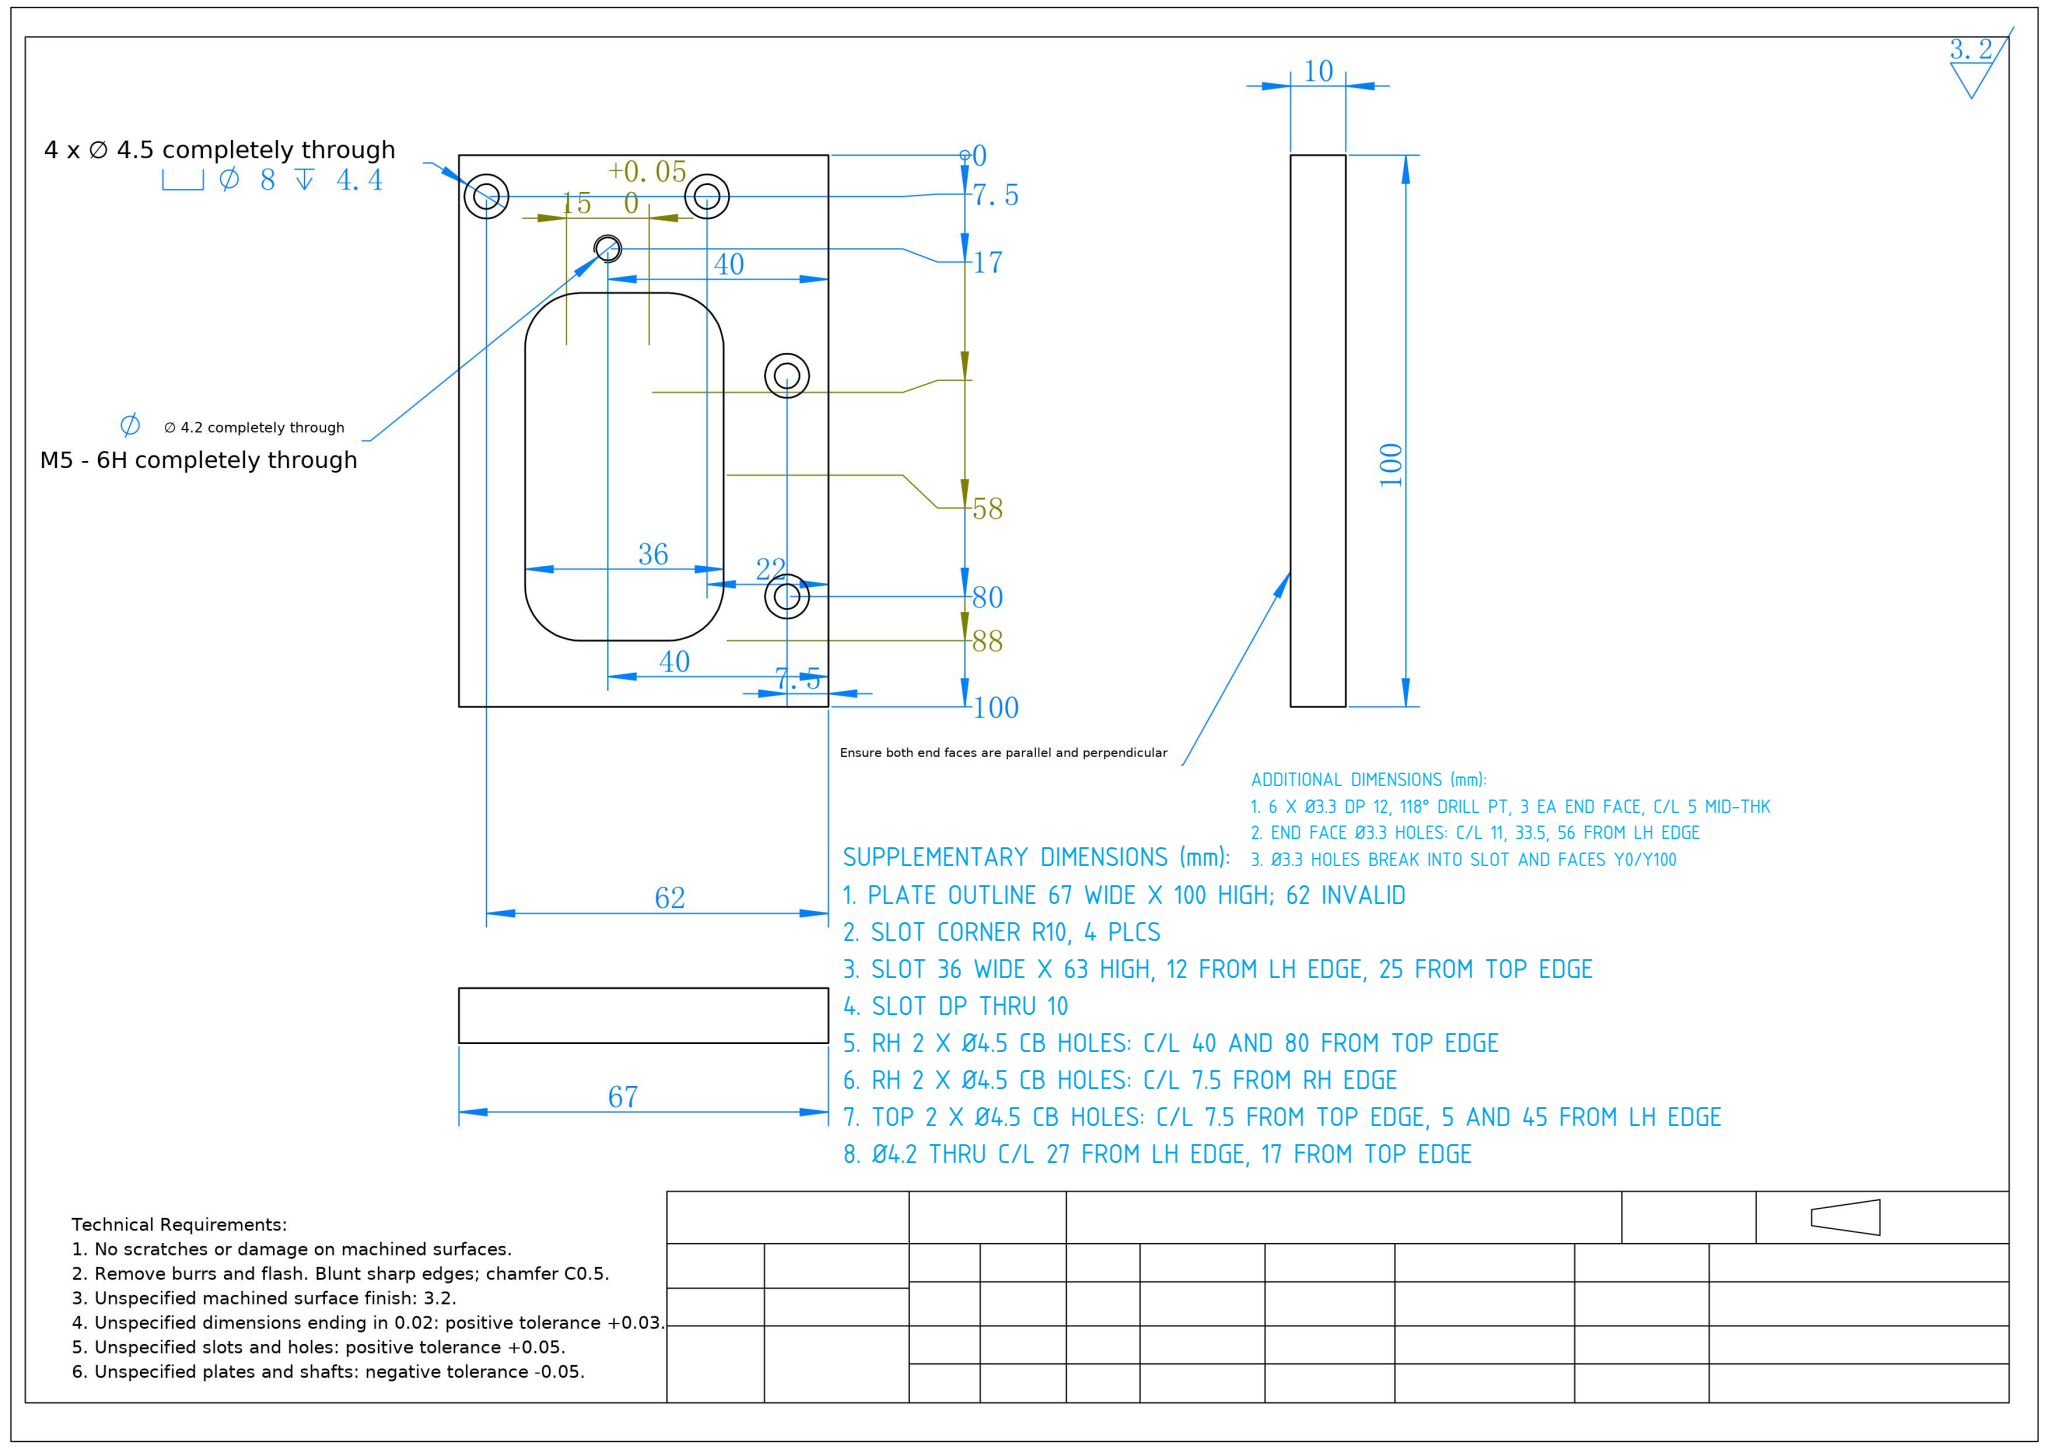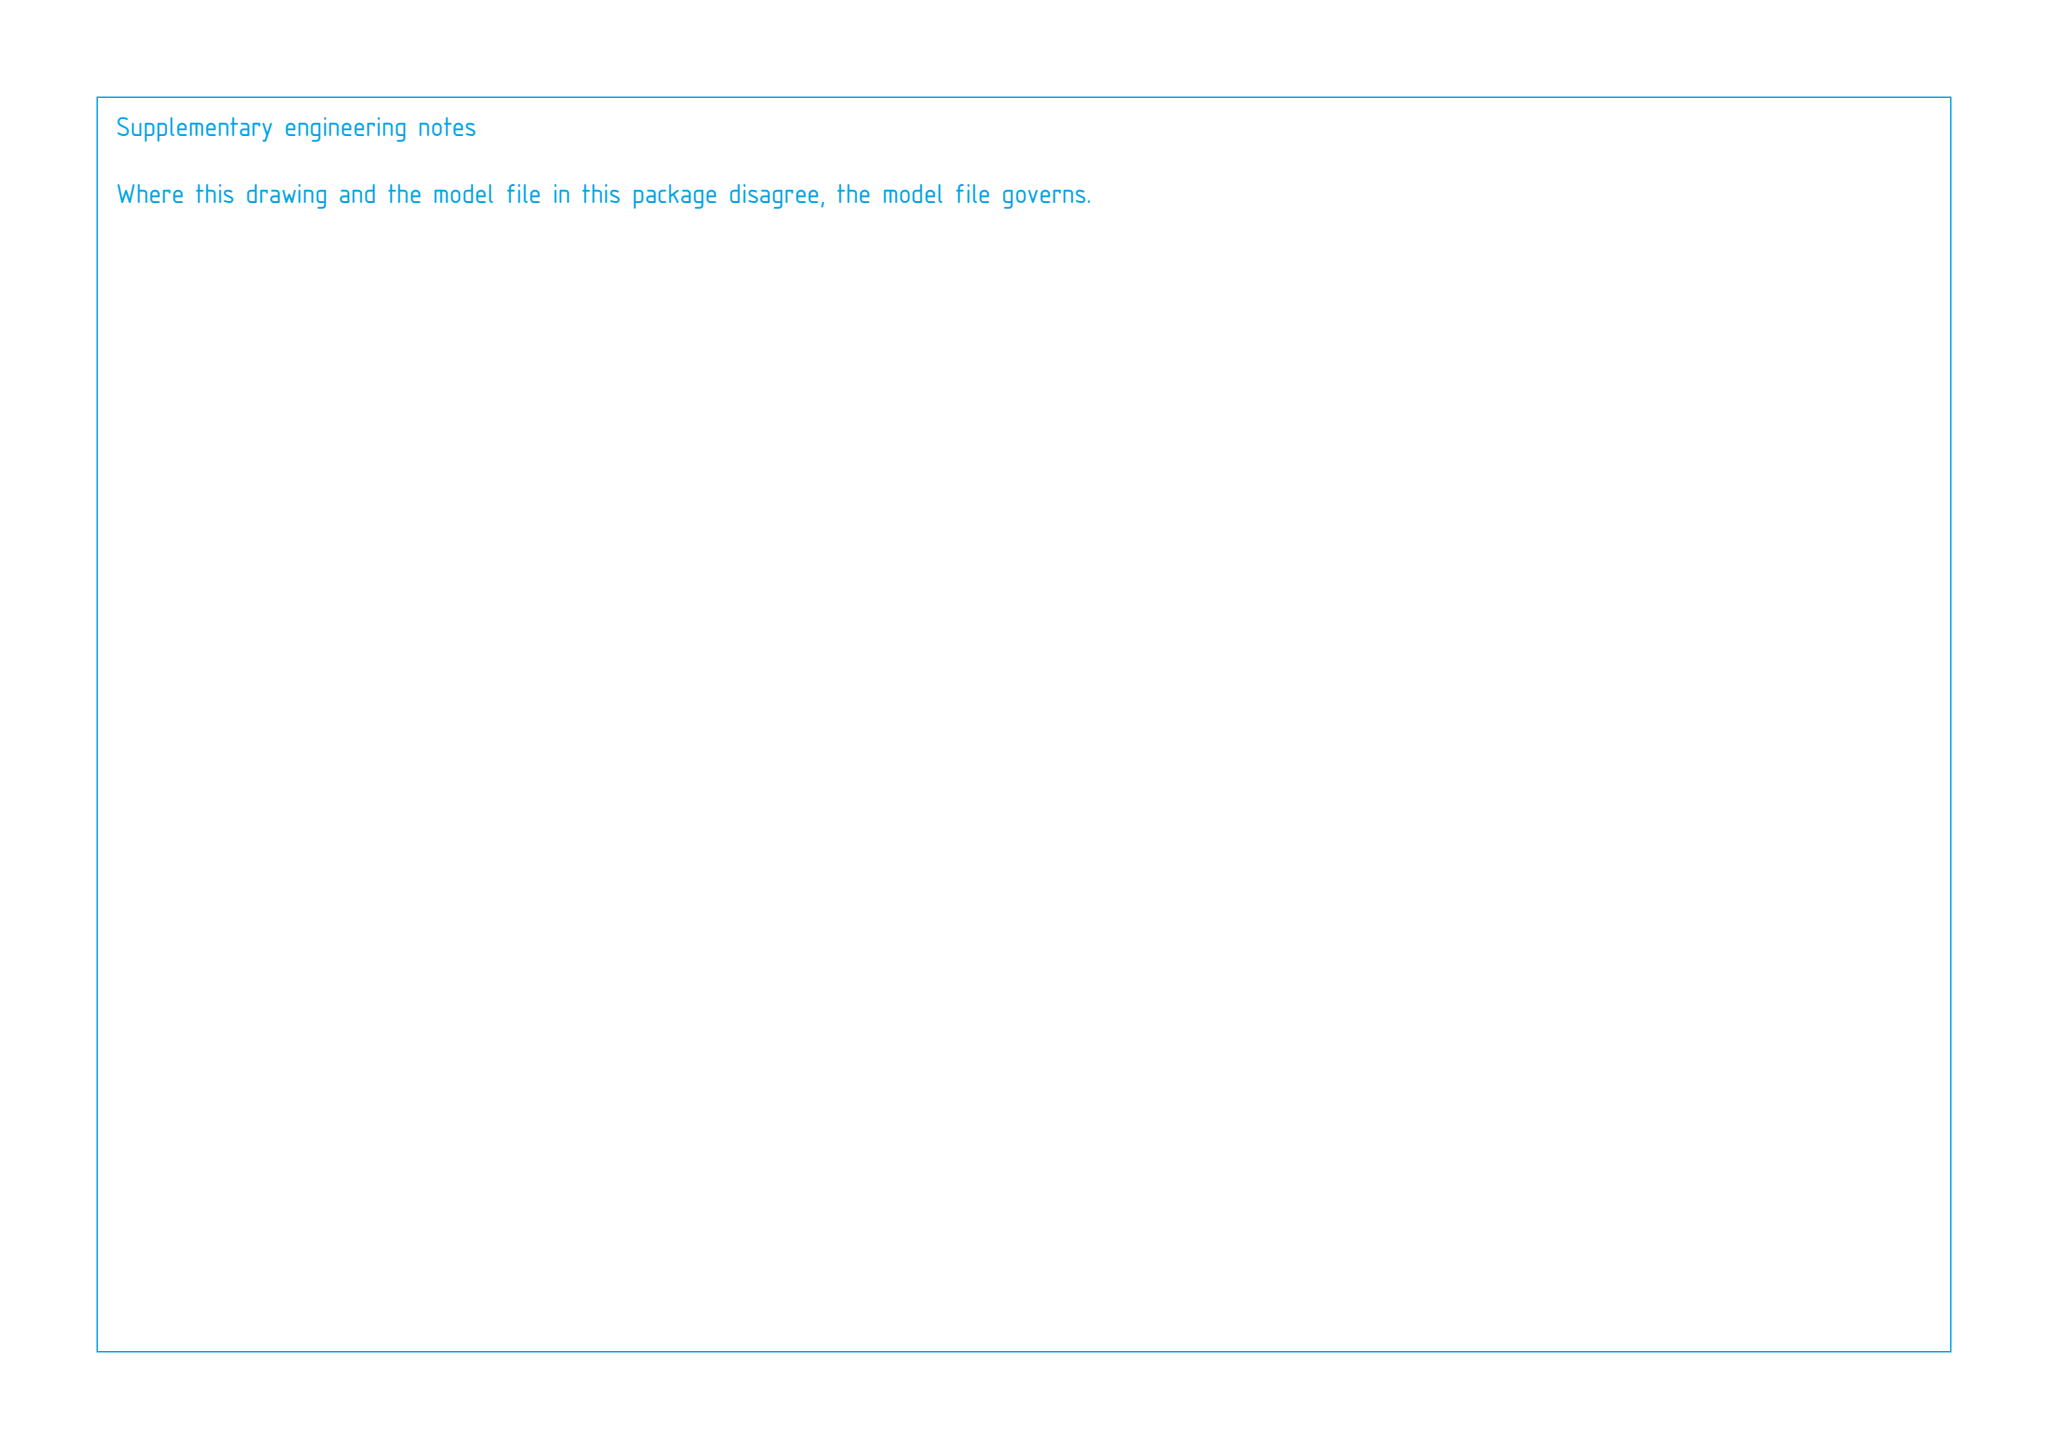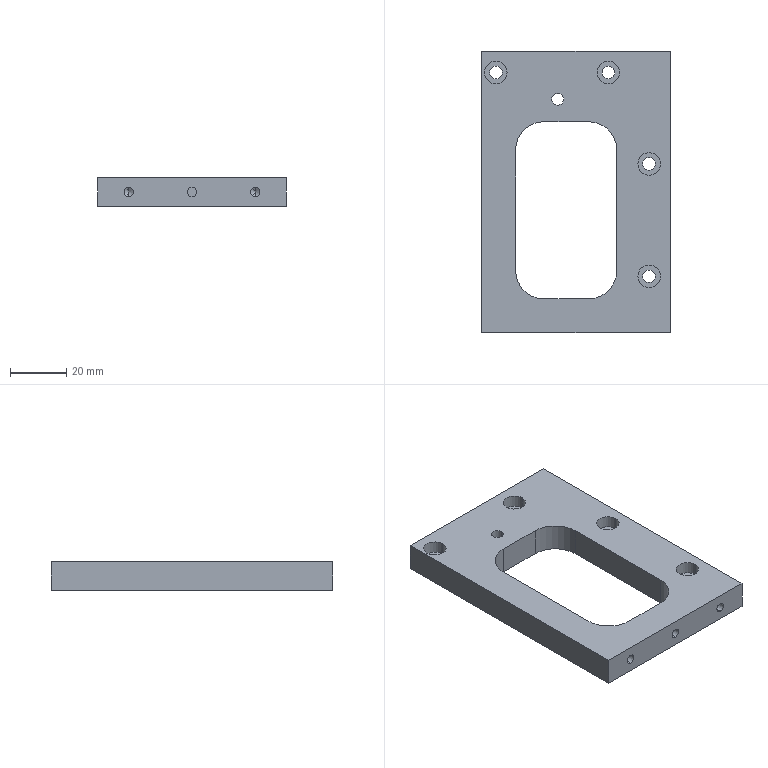Part | SolidWorks | mm | 1 solid | 46 faces | box 67 x 100 x 10 mm | volume 43485 mm3 | cylinder 28 | plane 14 | cone 4 | commonest cylinder face diameters 8 x8 4.5 x8 3.3 x6 20 x4 4.2 x2
build123d program:
from build123d import *

# Parameters (mm, degrees)
SKETCH1_W                                       = 67
SKETCH1_H                                       = 100
BOSS_EXTRUDE1_DEPTH                             = 10
SKETCH2_W                                       = 36
SKETCH2_H                                       = 63
CUT_EXTRUDE1_DEPTH                              = 106.935
FILLET1_R                                       = 10
M4_HEX_SOCKET_HEAD_CAP_SCREW_CBORE1_D           = 4.5
M4_HEX_SOCKET_HEAD_CAP_SCREW_CBORE1_CBORE_D     = 8
M4_HEX_SOCKET_HEAD_CAP_SCREW_CBORE1_CBORE_DEPTH = 4.4
M4_TAPPED_HOLE1_D                               = 3.3
M4_TAPPED_HOLE1_DEPTH                           = 12
M4_TAPPED_HOLE1_TIP                             = 0.9914
M5_TAPPED_HOLE1_D                               = 4.2


with BuildPart() as part:
    # Sketch1 → Boss-Extrude1 (new body)
    with BuildSketch(Plane.XY):
        with Locations((0, 50)):
            Rectangle(SKETCH1_W, SKETCH1_H)
    extrude(amount=BOSS_EXTRUDE1_DEPTH)

    # Sketch2 → Cut-Extrude1 (cut, through all)
    with BuildSketch(Plane.XY.offset(10)):
        with Locations((-3.5, 43.5)):
            Rectangle(SKETCH2_W, SKETCH2_H)
    extrude(amount=-CUT_EXTRUDE1_DEPTH, mode=Mode.SUBTRACT)

    # Fillet1
    fillet1_edges = [part.edges().sort_by_distance(p)[0] for p in [
        (14.5, 75, 5),
        (14.5, 12, 5),
        (-21.5, 12, 5),
        (-21.5, 75, 5),
    ]]
    fillet(fillet1_edges, radius=FILLET1_R)

    # M4 Hex Socket Head Cap Screw CBORE1 (through all)
    with Locations(Plane.XY.offset(10)):
        with Locations((26, 60), (26, 20), (11.5, 92.5), (-28.5, 92.5)):
            CounterBoreHole(M4_HEX_SOCKET_HEAD_CAP_SCREW_CBORE1_D / 2, M4_HEX_SOCKET_HEAD_CAP_SCREW_CBORE1_CBORE_D / 2, M4_HEX_SOCKET_HEAD_CAP_SCREW_CBORE1_CBORE_DEPTH)

    # M4 Tapped Hole1
    with Locations(Plane(origin=(0, 0, 0), x_dir=(-1, 0, 0), z_dir=(0, -1, 0))):
        with Locations((-22.5, -5), (0, -5), (22.5, -5)):
            Hole(M4_TAPPED_HOLE1_D / 2, depth=M4_TAPPED_HOLE1_DEPTH)
            with Locations((0, 0, -(M4_TAPPED_HOLE1_DEPTH + M4_TAPPED_HOLE1_TIP / 2))):  # 118° drill point
                Cone(0, M4_TAPPED_HOLE1_D / 2, M4_TAPPED_HOLE1_TIP, mode=Mode.SUBTRACT)

    # M5 Tapped Hole1 (through all)
    with Locations(Plane.XY.offset(10)):
        with Locations((-6.5, 83)):
            Hole(M5_TAPPED_HOLE1_D / 2)


solid = part.part